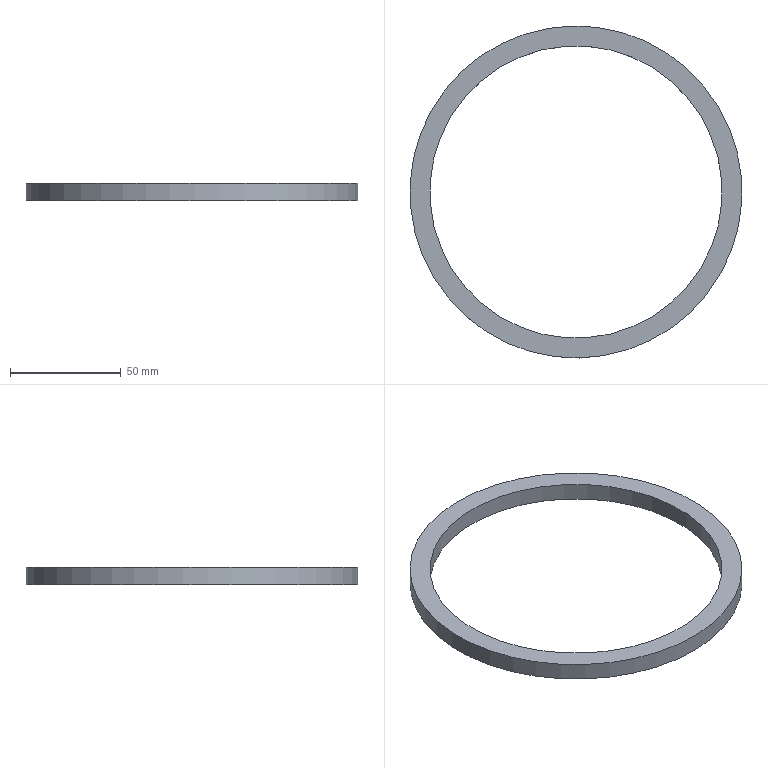Component | NX | CH3404-9 | 1 solid | 4 faces | box 150 x 150 x 8 mm | volume 31893 mm3 | cylinder 2 | plane 2 | commonest cylinder face diameters 150 x1 132 x1
STEP:
#1=CARTESIAN_POINT('',(0.,0.,0.));
#2=DIRECTION('',(0.,0.,1.));
#3=DIRECTION('',(1.,0.,0.));
#4=AXIS2_PLACEMENT_3D('',#1,#2,#3);
#5=CARTESIAN_POINT('',(-68.749,-28.623,-1500.3));
#6=VERTEX_POINT('',#5);
#7=CARTESIAN_POINT('',(0.5308,0.1057,-1500.3));
#8=DIRECTION('',(0.,0.,-1.));
#9=DIRECTION('',(-0.9237,-0.383,0.));
#10=AXIS2_PLACEMENT_3D('',#7,#8,#9);
#11=CIRCLE('',#10,75.);
#12=CARTESIAN_POINT('',(0.5308,0.1057,-1500.3));
#13=DIRECTION('',(0.,0.,1.));
#14=DIRECTION('',(0.9237,0.383,0.));
#15=AXIS2_PLACEMENT_3D('',#12,#13,#14);
#16=CYLINDRICAL_SURFACE('',#15,75.);
#17=CARTESIAN_POINT('',(9.425,0.));
#18=DIRECTION('',(-1.,0.));
#19=VECTOR('',#18,1.);
#20=LINE('',#17,#19);
#21=(GEOMETRIC_REPRESENTATION_CONTEXT(2)PARAMETRIC_REPRESENTATION_CONTEXT()REPRESENTATION_CONTEXT('',''));
#22=DEFINITIONAL_REPRESENTATION('',(#20),#21);
#23=PCURVE('',#16,#22);
#24=CARTESIAN_POINT('',(0.5308,0.1057,-1500.3));
#25=DIRECTION('',(0.,0.,-1.));
#26=DIRECTION('',(-0.9237,-0.383,0.));
#27=AXIS2_PLACEMENT_3D('',#24,#25,#26);
#28=PLANE('',#27);
#29=CARTESIAN_POINT('',(0.,0.));
#30=DIRECTION('',(1.,0.));
#31=AXIS2_PLACEMENT_2D('',#29,#30);
#32=CIRCLE('',#31,75.);
#33=(GEOMETRIC_REPRESENTATION_CONTEXT(2)PARAMETRIC_REPRESENTATION_CONTEXT()REPRESENTATION_CONTEXT('',''));
#34=DEFINITIONAL_REPRESENTATION('',(#32),#33);
#35=PCURVE('',#28,#34);
#36=SURFACE_CURVE('',#11,(#23,#35),.PCURVE_S1.);
#37=EDGE_CURVE('',#6,#6,#36,.T.);
#38=ORIENTED_EDGE('',*,*,#37,.F.);
#39=CARTESIAN_POINT('',(-68.749,-28.623,-1492.3));
#40=VERTEX_POINT('',#39);
#41=CARTESIAN_POINT('',(-68.749,-28.623,-1500.3));
#42=CARTESIAN_POINT('',(-68.749,-28.623,-1492.3));
#43=B_SPLINE_CURVE_WITH_KNOTS('',1,(#41,#42),.UNSPECIFIED.,.F.,.F.,(2,2),(0.,8.),.PIECEWISE_BEZIER_KNOTS.);
#44=CARTESIAN_POINT('',(9.425,0.));
#45=DIRECTION('',(0.,1.));
#46=VECTOR('',#45,1.);
#47=LINE('',#44,#46);
#48=(GEOMETRIC_REPRESENTATION_CONTEXT(2)PARAMETRIC_REPRESENTATION_CONTEXT()REPRESENTATION_CONTEXT('',''));
#49=DEFINITIONAL_REPRESENTATION('',(#47),#48);
#50=PCURVE('',#16,#49);
#51=CARTESIAN_POINT('',(3.142,0.));
#52=DIRECTION('',(0.,1.));
#53=VECTOR('',#52,1.);
#54=LINE('',#51,#53);
#55=(GEOMETRIC_REPRESENTATION_CONTEXT(2)PARAMETRIC_REPRESENTATION_CONTEXT()REPRESENTATION_CONTEXT('',''));
#56=DEFINITIONAL_REPRESENTATION('',(#54),#55);
#57=PCURVE('',#16,#56);
#58=SEAM_CURVE('',#43,(#50,#57),.PCURVE_S1.);
#59=EDGE_CURVE('',#6,#40,#58,.T.);
#60=ORIENTED_EDGE('',*,*,#59,.T.);
#61=CARTESIAN_POINT('',(0.5308,0.1057,-1492.3));
#62=DIRECTION('',(0.,0.,-1.));
#63=DIRECTION('',(-0.9237,-0.383,0.));
#64=AXIS2_PLACEMENT_3D('',#61,#62,#63);
#65=CIRCLE('',#64,75.);
#66=CARTESIAN_POINT('',(9.425,8.));
#67=DIRECTION('',(-1.,0.));
#68=VECTOR('',#67,1.);
#69=LINE('',#66,#68);
#70=(GEOMETRIC_REPRESENTATION_CONTEXT(2)PARAMETRIC_REPRESENTATION_CONTEXT()REPRESENTATION_CONTEXT('',''));
#71=DEFINITIONAL_REPRESENTATION('',(#69),#70);
#72=PCURVE('',#16,#71);
#73=CARTESIAN_POINT('',(0.5308,0.1057,-1492.3));
#74=DIRECTION('',(0.,0.,-1.));
#75=DIRECTION('',(-0.9237,-0.383,0.));
#76=AXIS2_PLACEMENT_3D('',#73,#74,#75);
#77=PLANE('',#76);
#78=CARTESIAN_POINT('',(0.,0.));
#79=DIRECTION('',(1.,0.));
#80=AXIS2_PLACEMENT_2D('',#78,#79);
#81=CIRCLE('',#80,75.);
#82=(GEOMETRIC_REPRESENTATION_CONTEXT(2)PARAMETRIC_REPRESENTATION_CONTEXT()REPRESENTATION_CONTEXT('',''));
#83=DEFINITIONAL_REPRESENTATION('',(#81),#82);
#84=PCURVE('',#77,#83);
#85=SURFACE_CURVE('',#65,(#72,#84),.PCURVE_S1.);
#86=EDGE_CURVE('',#40,#40,#85,.T.);
#87=ORIENTED_EDGE('',*,*,#86,.T.);
#88=ORIENTED_EDGE('',*,*,#59,.F.);
#89=EDGE_LOOP('',(#38,#60,#87,#88));
#90=FACE_BOUND('',#89,.T.);
#91=ADVANCED_FACE('',(#90),#16,.T.);
#92=CARTESIAN_POINT('',(-60.435,-25.176,-1500.3));
#93=VERTEX_POINT('',#92);
#94=CARTESIAN_POINT('',(0.5308,0.1057,-1500.3));
#95=DIRECTION('',(0.,0.,-1.));
#96=DIRECTION('',(-0.9237,-0.383,0.));
#97=AXIS2_PLACEMENT_3D('',#94,#95,#96);
#98=CIRCLE('',#97,66.);
#99=CARTESIAN_POINT('',(0.5308,0.1057,-1500.3));
#100=DIRECTION('',(0.,0.,1.));
#101=DIRECTION('',(0.9237,0.383,0.));
#102=AXIS2_PLACEMENT_3D('',#99,#100,#101);
#103=CYLINDRICAL_SURFACE('',#102,66.);
#104=CARTESIAN_POINT('',(9.425,0.));
#105=DIRECTION('',(-1.,0.));
#106=VECTOR('',#105,1.);
#107=LINE('',#104,#106);
#108=(GEOMETRIC_REPRESENTATION_CONTEXT(2)PARAMETRIC_REPRESENTATION_CONTEXT()REPRESENTATION_CONTEXT('',''));
#109=DEFINITIONAL_REPRESENTATION('',(#107),#108);
#110=PCURVE('',#103,#109);
#111=CARTESIAN_POINT('',(0.,0.));
#112=DIRECTION('',(1.,0.));
#113=AXIS2_PLACEMENT_2D('',#111,#112);
#114=CIRCLE('',#113,66.);
#115=(GEOMETRIC_REPRESENTATION_CONTEXT(2)PARAMETRIC_REPRESENTATION_CONTEXT()REPRESENTATION_CONTEXT('',''));
#116=DEFINITIONAL_REPRESENTATION('',(#114),#115);
#117=PCURVE('',#28,#116);
#118=SURFACE_CURVE('',#98,(#110,#117),.PCURVE_S1.);
#119=EDGE_CURVE('',#93,#93,#118,.T.);
#120=ORIENTED_EDGE('',*,*,#119,.F.);
#121=CARTESIAN_POINT('',(-60.435,-25.176,-1492.3));
#122=VERTEX_POINT('',#121);
#123=CARTESIAN_POINT('',(-60.435,-25.176,-1500.3));
#124=CARTESIAN_POINT('',(-60.435,-25.176,-1492.3));
#125=B_SPLINE_CURVE_WITH_KNOTS('',1,(#123,#124),.UNSPECIFIED.,.F.,.F.,(2,2),(0.,8.),.PIECEWISE_BEZIER_KNOTS.);
#126=CARTESIAN_POINT('',(9.425,0.));
#127=DIRECTION('',(0.,1.));
#128=VECTOR('',#127,1.);
#129=LINE('',#126,#128);
#130=(GEOMETRIC_REPRESENTATION_CONTEXT(2)PARAMETRIC_REPRESENTATION_CONTEXT()REPRESENTATION_CONTEXT('',''));
#131=DEFINITIONAL_REPRESENTATION('',(#129),#130);
#132=PCURVE('',#103,#131);
#133=CARTESIAN_POINT('',(3.142,0.));
#134=DIRECTION('',(0.,1.));
#135=VECTOR('',#134,1.);
#136=LINE('',#133,#135);
#137=(GEOMETRIC_REPRESENTATION_CONTEXT(2)PARAMETRIC_REPRESENTATION_CONTEXT()REPRESENTATION_CONTEXT('',''));
#138=DEFINITIONAL_REPRESENTATION('',(#136),#137);
#139=PCURVE('',#103,#138);
#140=SEAM_CURVE('',#125,(#132,#139),.PCURVE_S1.);
#141=EDGE_CURVE('',#93,#122,#140,.T.);
#142=ORIENTED_EDGE('',*,*,#141,.T.);
#143=CARTESIAN_POINT('',(0.5308,0.1057,-1492.3));
#144=DIRECTION('',(0.,0.,-1.));
#145=DIRECTION('',(-0.9237,-0.383,0.));
#146=AXIS2_PLACEMENT_3D('',#143,#144,#145);
#147=CIRCLE('',#146,66.);
#148=CARTESIAN_POINT('',(9.425,8.));
#149=DIRECTION('',(-1.,0.));
#150=VECTOR('',#149,1.);
#151=LINE('',#148,#150);
#152=(GEOMETRIC_REPRESENTATION_CONTEXT(2)PARAMETRIC_REPRESENTATION_CONTEXT()REPRESENTATION_CONTEXT('',''));
#153=DEFINITIONAL_REPRESENTATION('',(#151),#152);
#154=PCURVE('',#103,#153);
#155=CARTESIAN_POINT('',(0.,0.));
#156=DIRECTION('',(1.,0.));
#157=AXIS2_PLACEMENT_2D('',#155,#156);
#158=CIRCLE('',#157,66.);
#159=(GEOMETRIC_REPRESENTATION_CONTEXT(2)PARAMETRIC_REPRESENTATION_CONTEXT()REPRESENTATION_CONTEXT('',''));
#160=DEFINITIONAL_REPRESENTATION('',(#158),#159);
#161=PCURVE('',#77,#160);
#162=SURFACE_CURVE('',#147,(#154,#161),.PCURVE_S1.);
#163=EDGE_CURVE('',#122,#122,#162,.T.);
#164=ORIENTED_EDGE('',*,*,#163,.T.);
#165=ORIENTED_EDGE('',*,*,#141,.F.);
#166=EDGE_LOOP('',(#120,#142,#164,#165));
#167=FACE_BOUND('',#166,.F.);
#168=ADVANCED_FACE('',(#167),#103,.F.);
#169=ORIENTED_EDGE('',*,*,#37,.T.);
#170=EDGE_LOOP('',(#169));
#171=FACE_BOUND('',#170,.T.);
#172=ORIENTED_EDGE('',*,*,#119,.F.);
#173=EDGE_LOOP('',(#172));
#174=FACE_BOUND('',#173,.T.);
#175=ADVANCED_FACE('',(#171,#174),#28,.T.);
#176=ORIENTED_EDGE('',*,*,#86,.F.);
#177=EDGE_LOOP('',(#176));
#178=FACE_BOUND('',#177,.T.);
#179=ORIENTED_EDGE('',*,*,#163,.T.);
#180=EDGE_LOOP('',(#179));
#181=FACE_BOUND('',#180,.T.);
#182=ADVANCED_FACE('',(#178,#181),#77,.F.);
#183=CLOSED_SHELL('',(#91,#168,#175,#182));
#184=MANIFOLD_SOLID_BREP('',#183);
#185=(LENGTH_UNIT()NAMED_UNIT(*)SI_UNIT(.MILLI.,.METRE.));
#186=UNCERTAINTY_MEASURE_WITH_UNIT(LENGTH_MEASURE(0.00001),#185,'','');
#187=(NAMED_UNIT(*)PLANE_ANGLE_UNIT()SI_UNIT($,.RADIAN.));
#188=(NAMED_UNIT(*)SI_UNIT($,.STERADIAN.)SOLID_ANGLE_UNIT());
#189=(GEOMETRIC_REPRESENTATION_CONTEXT(3)GLOBAL_UNCERTAINTY_ASSIGNED_CONTEXT((#186))GLOBAL_UNIT_ASSIGNED_CONTEXT((#185,#187,#188))REPRESENTATION_CONTEXT('',''));
#190=ADVANCED_BREP_SHAPE_REPRESENTATION('',(#4,#184),#189);